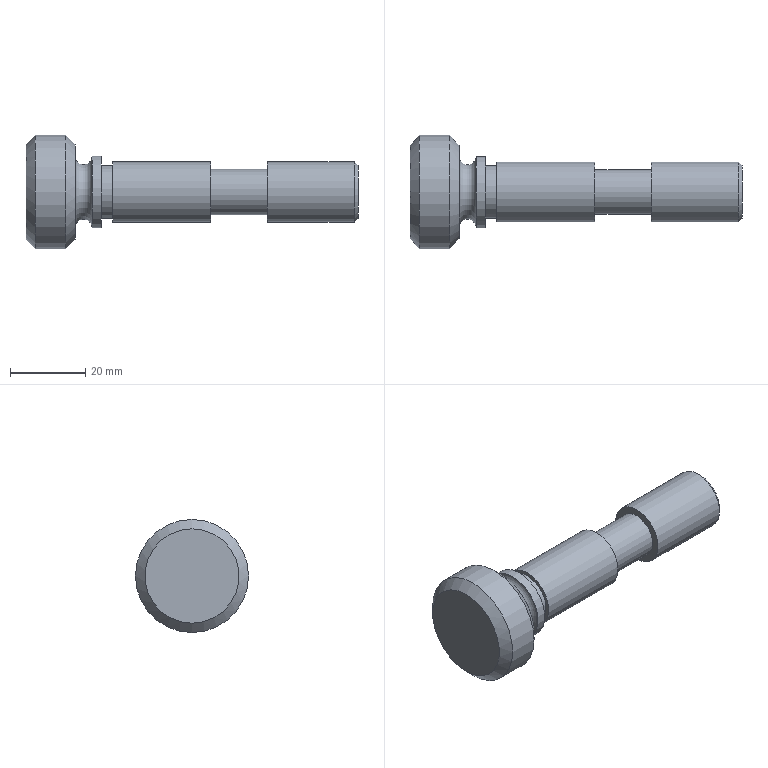Component | NX | SCREW_ROD | 1 solid | 17 faces | box 88 x 30 x 30 mm | volume 22378 mm3 | plane 7 | cylinder 6 | cone 3 | torus 1 | commonest cylinder face diameters 16 x2 12 x1 14 x1 19 x1 30 x1
STEP:
#1=CARTESIAN_POINT('',(0.,0.,0.));
#2=DIRECTION('',(0.,0.,1.));
#3=DIRECTION('',(1.,0.,0.));
#4=AXIS2_PLACEMENT_3D('',#1,#2,#3);
#5=CARTESIAN_POINT('',(-29.415,0.,-12.5));
#6=VERTEX_POINT('',#5);
#7=CARTESIAN_POINT('',(-29.415,0.,0.));
#8=DIRECTION('',(1.,0.,0.));
#9=DIRECTION('',(0.,0.,-1.));
#10=AXIS2_PLACEMENT_3D('',#7,#8,#9);
#11=CIRCLE('',#10,12.5);
#12=CARTESIAN_POINT('',(-29.415,0.,0.));
#13=DIRECTION('',(1.,0.,0.));
#14=DIRECTION('',(0.,0.,-1.));
#15=AXIS2_PLACEMENT_3D('',#12,#13,#14);
#16=PLANE('',#15);
#17=CARTESIAN_POINT('',(0.,0.));
#18=DIRECTION('',(1.,0.));
#19=AXIS2_PLACEMENT_2D('',#17,#18);
#20=CIRCLE('',#19,12.5);
#21=(GEOMETRIC_REPRESENTATION_CONTEXT(2)PARAMETRIC_REPRESENTATION_CONTEXT()REPRESENTATION_CONTEXT('',''));
#22=DEFINITIONAL_REPRESENTATION('',(#20),#21);
#23=PCURVE('',#16,#22);
#24=CARTESIAN_POINT('',(-29.415,0.,0.));
#25=DIRECTION('',(1.,0.,0.));
#26=DIRECTION('',(0.,0.,-1.));
#27=AXIS2_PLACEMENT_3D('',#24,#25,#26);
#28=CONICAL_SURFACE('',#27,12.5,0.7854);
#29=CARTESIAN_POINT('',(0.,0.));
#30=DIRECTION('',(1.,0.));
#31=VECTOR('',#30,1.);
#32=LINE('',#29,#31);
#33=(GEOMETRIC_REPRESENTATION_CONTEXT(2)PARAMETRIC_REPRESENTATION_CONTEXT()REPRESENTATION_CONTEXT('',''));
#34=DEFINITIONAL_REPRESENTATION('',(#32),#33);
#35=PCURVE('',#28,#34);
#36=SURFACE_CURVE('',#11,(#23,#35),.PCURVE_S1.);
#37=EDGE_CURVE('',#6,#6,#36,.T.);
#38=ORIENTED_EDGE('',*,*,#37,.F.);
#39=EDGE_LOOP('',(#38));
#40=FACE_BOUND('',#39,.T.);
#41=ADVANCED_FACE('',(#40),#16,.F.);
#42=CARTESIAN_POINT('',(58.585,0.,-7.));
#43=VERTEX_POINT('',#42);
#44=CARTESIAN_POINT('',(58.585,0.,0.));
#45=DIRECTION('',(1.,0.,0.));
#46=DIRECTION('',(0.,0.,-1.));
#47=AXIS2_PLACEMENT_3D('',#44,#45,#46);
#48=CIRCLE('',#47,7.);
#49=CARTESIAN_POINT('',(58.585,0.,0.));
#50=DIRECTION('',(1.,0.,0.));
#51=DIRECTION('',(0.,0.,-1.));
#52=AXIS2_PLACEMENT_3D('',#49,#50,#51);
#53=PLANE('',#52);
#54=CARTESIAN_POINT('',(0.,0.));
#55=DIRECTION('',(1.,0.));
#56=AXIS2_PLACEMENT_2D('',#54,#55);
#57=CIRCLE('',#56,7.);
#58=(GEOMETRIC_REPRESENTATION_CONTEXT(2)PARAMETRIC_REPRESENTATION_CONTEXT()REPRESENTATION_CONTEXT('',''));
#59=DEFINITIONAL_REPRESENTATION('',(#57),#58);
#60=PCURVE('',#53,#59);
#61=CARTESIAN_POINT('',(58.585,0.,0.));
#62=DIRECTION('',(-1.,0.,0.));
#63=DIRECTION('',(0.,0.,1.));
#64=AXIS2_PLACEMENT_3D('',#61,#62,#63);
#65=CONICAL_SURFACE('',#64,7.,0.7854);
#66=CARTESIAN_POINT('',(9.425,0.));
#67=DIRECTION('',(-1.,0.));
#68=VECTOR('',#67,1.);
#69=LINE('',#66,#68);
#70=(GEOMETRIC_REPRESENTATION_CONTEXT(2)PARAMETRIC_REPRESENTATION_CONTEXT()REPRESENTATION_CONTEXT('',''));
#71=DEFINITIONAL_REPRESENTATION('',(#69),#70);
#72=PCURVE('',#65,#71);
#73=SURFACE_CURVE('',#48,(#60,#72),.PCURVE_S1.);
#74=EDGE_CURVE('',#43,#43,#73,.T.);
#75=ORIENTED_EDGE('',*,*,#74,.T.);
#76=EDGE_LOOP('',(#75));
#77=FACE_BOUND('',#76,.T.);
#78=ADVANCED_FACE('',(#77),#53,.T.);
#79=CARTESIAN_POINT('',(57.585,0.,-8.));
#80=VERTEX_POINT('',#79);
#81=CARTESIAN_POINT('',(57.585,0.,0.));
#82=DIRECTION('',(-1.,0.,0.));
#83=DIRECTION('',(0.,0.,-1.));
#84=AXIS2_PLACEMENT_3D('',#81,#82,#83);
#85=CIRCLE('',#84,8.);
#86=CARTESIAN_POINT('',(58.585,0.,0.));
#87=DIRECTION('',(1.,0.,0.));
#88=DIRECTION('',(0.,0.,-1.));
#89=AXIS2_PLACEMENT_3D('',#86,#87,#88);
#90=CYLINDRICAL_SURFACE('',#89,8.);
#91=CARTESIAN_POINT('',(6.283,-1.));
#92=DIRECTION('',(-1.,0.));
#93=VECTOR('',#92,1.);
#94=LINE('',#91,#93);
#95=(GEOMETRIC_REPRESENTATION_CONTEXT(2)PARAMETRIC_REPRESENTATION_CONTEXT()REPRESENTATION_CONTEXT('',''));
#96=DEFINITIONAL_REPRESENTATION('',(#94),#95);
#97=PCURVE('',#90,#96);
#98=CARTESIAN_POINT('',(3.142,1.));
#99=DIRECTION('',(1.,0.));
#100=VECTOR('',#99,1.);
#101=LINE('',#98,#100);
#102=(GEOMETRIC_REPRESENTATION_CONTEXT(2)PARAMETRIC_REPRESENTATION_CONTEXT()REPRESENTATION_CONTEXT('',''));
#103=DEFINITIONAL_REPRESENTATION('',(#101),#102);
#104=PCURVE('',#65,#103);
#105=SURFACE_CURVE('',#85,(#97,#104),.PCURVE_S1.);
#106=EDGE_CURVE('',#80,#80,#105,.T.);
#107=ORIENTED_EDGE('',*,*,#106,.T.);
#108=CARTESIAN_POINT('',(34.585,0.,-8.));
#109=VERTEX_POINT('',#108);
#110=CARTESIAN_POINT('',(34.585,-0.,-8.));
#111=CARTESIAN_POINT('',(57.585,-0.,-8.));
#112=B_SPLINE_CURVE_WITH_KNOTS('',1,(#110,#111),.UNSPECIFIED.,.F.,.F.,(2,2),(-24.,-1.),.PIECEWISE_BEZIER_KNOTS.);
#113=CARTESIAN_POINT('',(0.,0.));
#114=DIRECTION('',(0.,1.));
#115=VECTOR('',#114,1.);
#116=LINE('',#113,#115);
#117=(GEOMETRIC_REPRESENTATION_CONTEXT(2)PARAMETRIC_REPRESENTATION_CONTEXT()REPRESENTATION_CONTEXT('',''));
#118=DEFINITIONAL_REPRESENTATION('',(#116),#117);
#119=PCURVE('',#90,#118);
#120=CARTESIAN_POINT('',(6.283,0.));
#121=DIRECTION('',(0.,1.));
#122=VECTOR('',#121,1.);
#123=LINE('',#120,#122);
#124=(GEOMETRIC_REPRESENTATION_CONTEXT(2)PARAMETRIC_REPRESENTATION_CONTEXT()REPRESENTATION_CONTEXT('',''));
#125=DEFINITIONAL_REPRESENTATION('',(#123),#124);
#126=PCURVE('',#90,#125);
#127=SEAM_CURVE('',#112,(#119,#126),.PCURVE_S1.);
#128=EDGE_CURVE('',#109,#80,#127,.T.);
#129=ORIENTED_EDGE('',*,*,#128,.F.);
#130=CARTESIAN_POINT('',(34.585,0.,0.));
#131=DIRECTION('',(1.,0.,0.));
#132=DIRECTION('',(0.,0.,-1.));
#133=AXIS2_PLACEMENT_3D('',#130,#131,#132);
#134=CIRCLE('',#133,8.);
#135=CARTESIAN_POINT('',(0.,-24.));
#136=DIRECTION('',(1.,0.));
#137=VECTOR('',#136,1.);
#138=LINE('',#135,#137);
#139=(GEOMETRIC_REPRESENTATION_CONTEXT(2)PARAMETRIC_REPRESENTATION_CONTEXT()REPRESENTATION_CONTEXT('',''));
#140=DEFINITIONAL_REPRESENTATION('',(#138),#139);
#141=PCURVE('',#90,#140);
#142=CARTESIAN_POINT('',(34.585,6.,0.));
#143=DIRECTION('',(1.,0.,0.));
#144=DIRECTION('',(0.,0.,-1.));
#145=AXIS2_PLACEMENT_3D('',#142,#143,#144);
#146=PLANE('',#145);
#147=CARTESIAN_POINT('',(0.,-6.));
#148=DIRECTION('',(1.,0.));
#149=AXIS2_PLACEMENT_2D('',#147,#148);
#150=CIRCLE('',#149,8.);
#151=(GEOMETRIC_REPRESENTATION_CONTEXT(2)PARAMETRIC_REPRESENTATION_CONTEXT()REPRESENTATION_CONTEXT('',''));
#152=DEFINITIONAL_REPRESENTATION('',(#150),#151);
#153=PCURVE('',#146,#152);
#154=SURFACE_CURVE('',#134,(#141,#153),.PCURVE_S1.);
#155=EDGE_CURVE('',#109,#109,#154,.T.);
#156=ORIENTED_EDGE('',*,*,#155,.T.);
#157=ORIENTED_EDGE('',*,*,#128,.T.);
#158=EDGE_LOOP('',(#107,#129,#156,#157));
#159=FACE_BOUND('',#158,.T.);
#160=ADVANCED_FACE('',(#159),#90,.T.);
#161=ORIENTED_EDGE('',*,*,#155,.F.);
#162=EDGE_LOOP('',(#161));
#163=FACE_BOUND('',#162,.T.);
#164=CARTESIAN_POINT('',(34.585,0.,-6.));
#165=VERTEX_POINT('',#164);
#166=CARTESIAN_POINT('',(34.585,0.,0.));
#167=DIRECTION('',(1.,0.,0.));
#168=DIRECTION('',(0.,0.,-1.));
#169=AXIS2_PLACEMENT_3D('',#166,#167,#168);
#170=CIRCLE('',#169,6.);
#171=CARTESIAN_POINT('',(0.,-6.));
#172=DIRECTION('',(1.,0.));
#173=AXIS2_PLACEMENT_2D('',#171,#172);
#174=CIRCLE('',#173,6.);
#175=(GEOMETRIC_REPRESENTATION_CONTEXT(2)PARAMETRIC_REPRESENTATION_CONTEXT()REPRESENTATION_CONTEXT('',''));
#176=DEFINITIONAL_REPRESENTATION('',(#174),#175);
#177=PCURVE('',#146,#176);
#178=CARTESIAN_POINT('',(58.585,0.,0.));
#179=DIRECTION('',(1.,0.,0.));
#180=DIRECTION('',(0.,0.,-1.));
#181=AXIS2_PLACEMENT_3D('',#178,#179,#180);
#182=CYLINDRICAL_SURFACE('',#181,6.);
#183=CARTESIAN_POINT('',(0.,-24.));
#184=DIRECTION('',(1.,0.));
#185=VECTOR('',#184,1.);
#186=LINE('',#183,#185);
#187=(GEOMETRIC_REPRESENTATION_CONTEXT(2)PARAMETRIC_REPRESENTATION_CONTEXT()REPRESENTATION_CONTEXT('',''));
#188=DEFINITIONAL_REPRESENTATION('',(#186),#187);
#189=PCURVE('',#182,#188);
#190=SURFACE_CURVE('',#170,(#177,#189),.PCURVE_S1.);
#191=EDGE_CURVE('',#165,#165,#190,.T.);
#192=ORIENTED_EDGE('',*,*,#191,.T.);
#193=EDGE_LOOP('',(#192));
#194=FACE_BOUND('',#193,.T.);
#195=ADVANCED_FACE('',(#163,#194),#146,.F.);
#196=ORIENTED_EDGE('',*,*,#191,.F.);
#197=CARTESIAN_POINT('',(19.585,0.,-6.));
#198=VERTEX_POINT('',#197);
#199=CARTESIAN_POINT('',(19.585,-0.,-6.));
#200=CARTESIAN_POINT('',(34.585,-0.,-6.));
#201=B_SPLINE_CURVE_WITH_KNOTS('',1,(#199,#200),.UNSPECIFIED.,.F.,.F.,(2,2),(-39.,-24.),.PIECEWISE_BEZIER_KNOTS.);
#202=CARTESIAN_POINT('',(0.,0.));
#203=DIRECTION('',(0.,1.));
#204=VECTOR('',#203,1.);
#205=LINE('',#202,#204);
#206=(GEOMETRIC_REPRESENTATION_CONTEXT(2)PARAMETRIC_REPRESENTATION_CONTEXT()REPRESENTATION_CONTEXT('',''));
#207=DEFINITIONAL_REPRESENTATION('',(#205),#206);
#208=PCURVE('',#182,#207);
#209=CARTESIAN_POINT('',(6.283,0.));
#210=DIRECTION('',(0.,1.));
#211=VECTOR('',#210,1.);
#212=LINE('',#209,#211);
#213=(GEOMETRIC_REPRESENTATION_CONTEXT(2)PARAMETRIC_REPRESENTATION_CONTEXT()REPRESENTATION_CONTEXT('',''));
#214=DEFINITIONAL_REPRESENTATION('',(#212),#213);
#215=PCURVE('',#182,#214);
#216=SEAM_CURVE('',#201,(#208,#215),.PCURVE_S1.);
#217=EDGE_CURVE('',#198,#165,#216,.T.);
#218=ORIENTED_EDGE('',*,*,#217,.F.);
#219=CARTESIAN_POINT('',(19.585,0.,0.));
#220=DIRECTION('',(1.,0.,0.));
#221=DIRECTION('',(0.,0.,-1.));
#222=AXIS2_PLACEMENT_3D('',#219,#220,#221);
#223=CIRCLE('',#222,6.);
#224=CARTESIAN_POINT('',(0.,-39.));
#225=DIRECTION('',(1.,0.));
#226=VECTOR('',#225,1.);
#227=LINE('',#224,#226);
#228=(GEOMETRIC_REPRESENTATION_CONTEXT(2)PARAMETRIC_REPRESENTATION_CONTEXT()REPRESENTATION_CONTEXT('',''));
#229=DEFINITIONAL_REPRESENTATION('',(#227),#228);
#230=PCURVE('',#182,#229);
#231=CARTESIAN_POINT('',(19.585,8.,0.));
#232=DIRECTION('',(-1.,0.,0.));
#233=DIRECTION('',(0.,0.,1.));
#234=AXIS2_PLACEMENT_3D('',#231,#232,#233);
#235=PLANE('',#234);
#236=CARTESIAN_POINT('',(-6.,-8.));
#237=CARTESIAN_POINT('',(-6.,2.392));
#238=CARTESIAN_POINT('',(3.,-2.804));
#239=CARTESIAN_POINT('',(12.,-8.));
#240=CARTESIAN_POINT('',(3.,-13.196));
#241=CARTESIAN_POINT('',(-6.,-18.392));
#242=CARTESIAN_POINT('',(-6.,-8.));
#243=(BOUNDED_CURVE()B_SPLINE_CURVE(2,(#236,#237,#238,#239,#240,#241,#242),.UNSPECIFIED.,.T.,.F.)B_SPLINE_CURVE_WITH_KNOTS((1,2,2,2,2,1),(-2.094,0.,2.094,4.189,6.283,8.378),.UNSPECIFIED.)CURVE()GEOMETRIC_REPRESENTATION_ITEM()RATIONAL_B_SPLINE_CURVE((1.,0.5,1.,0.5,1.,0.5,1.))REPRESENTATION_ITEM(''));
#244=(GEOMETRIC_REPRESENTATION_CONTEXT(2)PARAMETRIC_REPRESENTATION_CONTEXT()REPRESENTATION_CONTEXT('',''));
#245=DEFINITIONAL_REPRESENTATION('',(#243),#244);
#246=PCURVE('',#235,#245);
#247=SURFACE_CURVE('',#223,(#230,#246),.PCURVE_S1.);
#248=EDGE_CURVE('',#198,#198,#247,.T.);
#249=ORIENTED_EDGE('',*,*,#248,.T.);
#250=ORIENTED_EDGE('',*,*,#217,.T.);
#251=EDGE_LOOP('',(#196,#218,#249,#250));
#252=FACE_BOUND('',#251,.T.);
#253=ADVANCED_FACE('',(#252),#182,.T.);
#254=ORIENTED_EDGE('',*,*,#248,.F.);
#255=EDGE_LOOP('',(#254));
#256=FACE_BOUND('',#255,.T.);
#257=CARTESIAN_POINT('',(19.585,0.,-8.));
#258=VERTEX_POINT('',#257);
#259=CARTESIAN_POINT('',(19.585,0.,0.));
#260=DIRECTION('',(1.,0.,0.));
#261=DIRECTION('',(0.,0.,-1.));
#262=AXIS2_PLACEMENT_3D('',#259,#260,#261);
#263=CIRCLE('',#262,8.);
#264=CARTESIAN_POINT('',(-8.,-8.));
#265=CARTESIAN_POINT('',(-8.,5.856));
#266=CARTESIAN_POINT('',(4.,-1.072));
#267=CARTESIAN_POINT('',(16.,-8.));
#268=CARTESIAN_POINT('',(4.,-14.928));
#269=CARTESIAN_POINT('',(-8.,-21.856));
#270=CARTESIAN_POINT('',(-8.,-8.));
#271=(BOUNDED_CURVE()B_SPLINE_CURVE(2,(#264,#265,#266,#267,#268,#269,#270),.UNSPECIFIED.,.T.,.F.)B_SPLINE_CURVE_WITH_KNOTS((1,2,2,2,2,1),(-2.094,0.,2.094,4.189,6.283,8.378),.UNSPECIFIED.)CURVE()GEOMETRIC_REPRESENTATION_ITEM()RATIONAL_B_SPLINE_CURVE((1.,0.5,1.,0.5,1.,0.5,1.))REPRESENTATION_ITEM(''));
#272=(GEOMETRIC_REPRESENTATION_CONTEXT(2)PARAMETRIC_REPRESENTATION_CONTEXT()REPRESENTATION_CONTEXT('',''));
#273=DEFINITIONAL_REPRESENTATION('',(#271),#272);
#274=PCURVE('',#235,#273);
#275=CARTESIAN_POINT('',(58.585,0.,0.));
#276=DIRECTION('',(1.,0.,0.));
#277=DIRECTION('',(0.,0.,-1.));
#278=AXIS2_PLACEMENT_3D('',#275,#276,#277);
#279=CYLINDRICAL_SURFACE('',#278,8.);
#280=CARTESIAN_POINT('',(0.,-39.));
#281=DIRECTION('',(1.,0.));
#282=VECTOR('',#281,1.);
#283=LINE('',#280,#282);
#284=(GEOMETRIC_REPRESENTATION_CONTEXT(2)PARAMETRIC_REPRESENTATION_CONTEXT()REPRESENTATION_CONTEXT('',''));
#285=DEFINITIONAL_REPRESENTATION('',(#283),#284);
#286=PCURVE('',#279,#285);
#287=SURFACE_CURVE('',#263,(#274,#286),.PCURVE_S1.);
#288=EDGE_CURVE('',#258,#258,#287,.T.);
#289=ORIENTED_EDGE('',*,*,#288,.T.);
#290=EDGE_LOOP('',(#289));
#291=FACE_BOUND('',#290,.T.);
#292=ADVANCED_FACE('',(#256,#291),#235,.F.);
#293=ORIENTED_EDGE('',*,*,#288,.F.);
#294=CARTESIAN_POINT('',(-6.415,0.,-8.));
#295=VERTEX_POINT('',#294);
#296=CARTESIAN_POINT('',(-6.415,-0.,-8.));
#297=CARTESIAN_POINT('',(19.585,-0.,-8.));
#298=B_SPLINE_CURVE_WITH_KNOTS('',1,(#296,#297),.UNSPECIFIED.,.F.,.F.,(2,2),(-65.,-39.),.PIECEWISE_BEZIER_KNOTS.);
#299=CARTESIAN_POINT('',(0.,0.));
#300=DIRECTION('',(0.,1.));
#301=VECTOR('',#300,1.);
#302=LINE('',#299,#301);
#303=(GEOMETRIC_REPRESENTATION_CONTEXT(2)PARAMETRIC_REPRESENTATION_CONTEXT()REPRESENTATION_CONTEXT('',''));
#304=DEFINITIONAL_REPRESENTATION('',(#302),#303);
#305=PCURVE('',#279,#304);
#306=CARTESIAN_POINT('',(6.283,0.));
#307=DIRECTION('',(0.,1.));
#308=VECTOR('',#307,1.);
#309=LINE('',#306,#308);
#310=(GEOMETRIC_REPRESENTATION_CONTEXT(2)PARAMETRIC_REPRESENTATION_CONTEXT()REPRESENTATION_CONTEXT('',''));
#311=DEFINITIONAL_REPRESENTATION('',(#309),#310);
#312=PCURVE('',#279,#311);
#313=SEAM_CURVE('',#298,(#305,#312),.PCURVE_S1.);
#314=EDGE_CURVE('',#295,#258,#313,.T.);
#315=ORIENTED_EDGE('',*,*,#314,.F.);
#316=CARTESIAN_POINT('',(-6.415,0.,0.));
#317=DIRECTION('',(1.,0.,0.));
#318=DIRECTION('',(0.,0.,-1.));
#319=AXIS2_PLACEMENT_3D('',#316,#317,#318);
#320=CIRCLE('',#319,8.);
#321=CARTESIAN_POINT('',(0.,-65.));
#322=DIRECTION('',(1.,0.));
#323=VECTOR('',#322,1.);
#324=LINE('',#321,#323);
#325=(GEOMETRIC_REPRESENTATION_CONTEXT(2)PARAMETRIC_REPRESENTATION_CONTEXT()REPRESENTATION_CONTEXT('',''));
#326=DEFINITIONAL_REPRESENTATION('',(#324),#325);
#327=PCURVE('',#279,#326);
#328=CARTESIAN_POINT('',(-6.415,7.,0.));
#329=DIRECTION('',(1.,0.,0.));
#330=DIRECTION('',(0.,0.,-1.));
#331=AXIS2_PLACEMENT_3D('',#328,#329,#330);
#332=PLANE('',#331);
#333=CARTESIAN_POINT('',(0.,-7.));
#334=DIRECTION('',(1.,0.));
#335=AXIS2_PLACEMENT_2D('',#333,#334);
#336=CIRCLE('',#335,8.);
#337=(GEOMETRIC_REPRESENTATION_CONTEXT(2)PARAMETRIC_REPRESENTATION_CONTEXT()REPRESENTATION_CONTEXT('',''));
#338=DEFINITIONAL_REPRESENTATION('',(#336),#337);
#339=PCURVE('',#332,#338);
#340=SURFACE_CURVE('',#320,(#327,#339),.PCURVE_S1.);
#341=EDGE_CURVE('',#295,#295,#340,.T.);
#342=ORIENTED_EDGE('',*,*,#341,.T.);
#343=ORIENTED_EDGE('',*,*,#314,.T.);
#344=EDGE_LOOP('',(#293,#315,#342,#343));
#345=FACE_BOUND('',#344,.T.);
#346=ADVANCED_FACE('',(#345),#279,.T.);
#347=ORIENTED_EDGE('',*,*,#341,.F.);
#348=EDGE_LOOP('',(#347));
#349=FACE_BOUND('',#348,.T.);
#350=CARTESIAN_POINT('',(-6.415,0.,-7.));
#351=VERTEX_POINT('',#350);
#352=CARTESIAN_POINT('',(-6.415,0.,0.));
#353=DIRECTION('',(1.,0.,0.));
#354=DIRECTION('',(0.,0.,-1.));
#355=AXIS2_PLACEMENT_3D('',#352,#353,#354);
#356=CIRCLE('',#355,7.);
#357=CARTESIAN_POINT('',(0.,-7.));
#358=DIRECTION('',(1.,0.));
#359=AXIS2_PLACEMENT_2D('',#357,#358);
#360=CIRCLE('',#359,7.);
#361=(GEOMETRIC_REPRESENTATION_CONTEXT(2)PARAMETRIC_REPRESENTATION_CONTEXT()REPRESENTATION_CONTEXT('',''));
#362=DEFINITIONAL_REPRESENTATION('',(#360),#361);
#363=PCURVE('',#332,#362);
#364=CARTESIAN_POINT('',(58.585,0.,0.));
#365=DIRECTION('',(1.,0.,0.));
#366=DIRECTION('',(0.,0.,-1.));
#367=AXIS2_PLACEMENT_3D('',#364,#365,#366);
#368=CYLINDRICAL_SURFACE('',#367,7.);
#369=CARTESIAN_POINT('',(0.,-65.));
#370=DIRECTION('',(1.,0.));
#371=VECTOR('',#370,1.);
#372=LINE('',#369,#371);
#373=(GEOMETRIC_REPRESENTATION_CONTEXT(2)PARAMETRIC_REPRESENTATION_CONTEXT()REPRESENTATION_CONTEXT('',''));
#374=DEFINITIONAL_REPRESENTATION('',(#372),#373);
#375=PCURVE('',#368,#374);
#376=SURFACE_CURVE('',#356,(#363,#375),.PCURVE_S1.);
#377=EDGE_CURVE('',#351,#351,#376,.T.);
#378=ORIENTED_EDGE('',*,*,#377,.T.);
#379=EDGE_LOOP('',(#378));
#380=FACE_BOUND('',#379,.T.);
#381=ADVANCED_FACE('',(#349,#380),#332,.F.);
#382=ORIENTED_EDGE('',*,*,#377,.F.);
#383=CARTESIAN_POINT('',(-9.415,0.,-7.));
#384=VERTEX_POINT('',#383);
#385=CARTESIAN_POINT('',(-9.415,-0.,-7.));
#386=CARTESIAN_POINT('',(-6.415,-0.,-7.));
#387=B_SPLINE_CURVE_WITH_KNOTS('',1,(#385,#386),.UNSPECIFIED.,.F.,.F.,(2,2),(-68.,-65.),.PIECEWISE_BEZIER_KNOTS.);
#388=CARTESIAN_POINT('',(0.,0.));
#389=DIRECTION('',(0.,1.));
#390=VECTOR('',#389,1.);
#391=LINE('',#388,#390);
#392=(GEOMETRIC_REPRESENTATION_CONTEXT(2)PARAMETRIC_REPRESENTATION_CONTEXT()REPRESENTATION_CONTEXT('',''));
#393=DEFINITIONAL_REPRESENTATION('',(#391),#392);
#394=PCURVE('',#368,#393);
#395=CARTESIAN_POINT('',(6.283,0.));
#396=DIRECTION('',(0.,1.));
#397=VECTOR('',#396,1.);
#398=LINE('',#395,#397);
#399=(GEOMETRIC_REPRESENTATION_CONTEXT(2)PARAMETRIC_REPRESENTATION_CONTEXT()REPRESENTATION_CONTEXT('',''));
#400=DEFINITIONAL_REPRESENTATION('',(#398),#399);
#401=PCURVE('',#368,#400);
#402=SEAM_CURVE('',#387,(#394,#401),.PCURVE_S1.);
#403=EDGE_CURVE('',#384,#351,#402,.T.);
#404=ORIENTED_EDGE('',*,*,#403,.F.);
#405=CARTESIAN_POINT('',(-9.415,0.,0.));
#406=DIRECTION('',(1.,0.,0.));
#407=DIRECTION('',(0.,0.,-1.));
#408=AXIS2_PLACEMENT_3D('',#405,#406,#407);
#409=CIRCLE('',#408,7.);
#410=CARTESIAN_POINT('',(0.,-68.));
#411=DIRECTION('',(1.,0.));
#412=VECTOR('',#411,1.);
#413=LINE('',#410,#412);
#414=(GEOMETRIC_REPRESENTATION_CONTEXT(2)PARAMETRIC_REPRESENTATION_CONTEXT()REPRESENTATION_CONTEXT('',''));
#415=DEFINITIONAL_REPRESENTATION('',(#413),#414);
#416=PCURVE('',#368,#415);
#417=CARTESIAN_POINT('',(-9.415,9.5,0.));
#418=DIRECTION('',(-1.,0.,0.));
#419=DIRECTION('',(0.,0.,1.));
#420=AXIS2_PLACEMENT_3D('',#417,#418,#419);
#421=PLANE('',#420);
#422=CARTESIAN_POINT('',(-7.,-9.5));
#423=CARTESIAN_POINT('',(-7.,2.624));
#424=CARTESIAN_POINT('',(3.5,-3.438));
#425=CARTESIAN_POINT('',(14.,-9.5));
#426=CARTESIAN_POINT('',(3.5,-15.562));
#427=CARTESIAN_POINT('',(-7.,-21.624));
#428=CARTESIAN_POINT('',(-7.,-9.5));
#429=(BOUNDED_CURVE()B_SPLINE_CURVE(2,(#422,#423,#424,#425,#426,#427,#428),.UNSPECIFIED.,.T.,.F.)B_SPLINE_CURVE_WITH_KNOTS((1,2,2,2,2,1),(-2.094,0.,2.094,4.189,6.283,8.378),.UNSPECIFIED.)CURVE()GEOMETRIC_REPRESENTATION_ITEM()RATIONAL_B_SPLINE_CURVE((1.,0.5,1.,0.5,1.,0.5,1.))REPRESENTATION_ITEM(''));
#430=(GEOMETRIC_REPRESENTATION_CONTEXT(2)PARAMETRIC_REPRESENTATION_CONTEXT()REPRESENTATION_CONTEXT('',''));
#431=DEFINITIONAL_REPRESENTATION('',(#429),#430);
#432=PCURVE('',#421,#431);
#433=SURFACE_CURVE('',#409,(#416,#432),.PCURVE_S1.);
#434=EDGE_CURVE('',#384,#384,#433,.T.);
#435=ORIENTED_EDGE('',*,*,#434,.T.);
#436=ORIENTED_EDGE('',*,*,#403,.T.);
#437=EDGE_LOOP('',(#382,#404,#435,#436));
#438=FACE_BOUND('',#437,.T.);
#439=ADVANCED_FACE('',(#438),#368,.T.);
#440=ORIENTED_EDGE('',*,*,#434,.F.);
#441=EDGE_LOOP('',(#440));
#442=FACE_BOUND('',#441,.T.);
#443=CARTESIAN_POINT('',(-9.415,0.,-9.5));
#444=VERTEX_POINT('',#443);
#445=CARTESIAN_POINT('',(-9.415,0.,0.));
#446=DIRECTION('',(1.,0.,0.));
#447=DIRECTION('',(0.,0.,-1.));
#448=AXIS2_PLACEMENT_3D('',#445,#446,#447);
#449=CIRCLE('',#448,9.5);
#450=CARTESIAN_POINT('',(-9.5,-9.5));
#451=CARTESIAN_POINT('',(-9.5,6.954));
#452=CARTESIAN_POINT('',(4.75,-1.273));
#453=CARTESIAN_POINT('',(19.,-9.5));
#454=CARTESIAN_POINT('',(4.75,-17.727));
#455=CARTESIAN_POINT('',(-9.5,-25.954));
#456=CARTESIAN_POINT('',(-9.5,-9.5));
#457=(BOUNDED_CURVE()B_SPLINE_CURVE(2,(#450,#451,#452,#453,#454,#455,#456),.UNSPECIFIED.,.T.,.F.)B_SPLINE_CURVE_WITH_KNOTS((1,2,2,2,2,1),(-2.094,0.,2.094,4.189,6.283,8.378),.UNSPECIFIED.)CURVE()GEOMETRIC_REPRESENTATION_ITEM()RATIONAL_B_SPLINE_CURVE((1.,0.5,1.,0.5,1.,0.5,1.))REPRESENTATION_ITEM(''));
#458=(GEOMETRIC_REPRESENTATION_CONTEXT(2)PARAMETRIC_REPRESENTATION_CONTEXT()REPRESENTATION_CONTEXT('',''));
#459=DEFINITIONAL_REPRESENTATION('',(#457),#458);
#460=PCURVE('',#421,#459);
#461=CARTESIAN_POINT('',(58.585,0.,0.));
#462=DIRECTION('',(1.,0.,0.));
#463=DIRECTION('',(0.,0.,-1.));
#464=AXIS2_PLACEMENT_3D('',#461,#462,#463);
#465=CYLINDRICAL_SURFACE('',#464,9.5);
#466=CARTESIAN_POINT('',(0.,-68.));
#467=DIRECTION('',(1.,0.));
#468=VECTOR('',#467,1.);
#469=LINE('',#466,#468);
#470=(GEOMETRIC_REPRESENTATION_CONTEXT(2)PARAMETRIC_REPRESENTATION_CONTEXT()REPRESENTATION_CONTEXT('',''));
#471=DEFINITIONAL_REPRESENTATION('',(#469),#470);
#472=PCURVE('',#465,#471);
#473=SURFACE_CURVE('',#449,(#460,#472),.PCURVE_S1.);
#474=EDGE_CURVE('',#444,#444,#473,.T.);
#475=ORIENTED_EDGE('',*,*,#474,.T.);
#476=EDGE_LOOP('',(#475));
#477=FACE_BOUND('',#476,.T.);
#478=ADVANCED_FACE('',(#442,#477),#421,.F.);
#479=ORIENTED_EDGE('',*,*,#474,.F.);
#480=CARTESIAN_POINT('',(-11.915,0.,-9.5));
#481=VERTEX_POINT('',#480);
#482=CARTESIAN_POINT('',(-11.915,-0.,-9.5));
#483=CARTESIAN_POINT('',(-9.415,-0.,-9.5));
#484=B_SPLINE_CURVE_WITH_KNOTS('',1,(#482,#483),.UNSPECIFIED.,.F.,.F.,(2,2),(-70.5,-68.),.PIECEWISE_BEZIER_KNOTS.);
#485=CARTESIAN_POINT('',(0.,0.));
#486=DIRECTION('',(0.,1.));
#487=VECTOR('',#486,1.);
#488=LINE('',#485,#487);
#489=(GEOMETRIC_REPRESENTATION_CONTEXT(2)PARAMETRIC_REPRESENTATION_CONTEXT()REPRESENTATION_CONTEXT('',''));
#490=DEFINITIONAL_REPRESENTATION('',(#488),#489);
#491=PCURVE('',#465,#490);
#492=CARTESIAN_POINT('',(6.283,0.));
#493=DIRECTION('',(0.,1.));
#494=VECTOR('',#493,1.);
#495=LINE('',#492,#494);
#496=(GEOMETRIC_REPRESENTATION_CONTEXT(2)PARAMETRIC_REPRESENTATION_CONTEXT()REPRESENTATION_CONTEXT('',''));
#497=DEFINITIONAL_REPRESENTATION('',(#495),#496);
#498=PCURVE('',#465,#497);
#499=SEAM_CURVE('',#484,(#491,#498),.PCURVE_S1.);
#500=EDGE_CURVE('',#481,#444,#499,.T.);
#501=ORIENTED_EDGE('',*,*,#500,.F.);
#502=CARTESIAN_POINT('',(-11.915,0.,0.));
#503=DIRECTION('',(1.,0.,0.));
#504=DIRECTION('',(0.,0.,-1.));
#505=AXIS2_PLACEMENT_3D('',#502,#503,#504);
#506=CIRCLE('',#505,9.5);
#507=CARTESIAN_POINT('',(0.,-70.5));
#508=DIRECTION('',(1.,0.));
#509=VECTOR('',#508,1.);
#510=LINE('',#507,#509);
#511=(GEOMETRIC_REPRESENTATION_CONTEXT(2)PARAMETRIC_REPRESENTATION_CONTEXT()REPRESENTATION_CONTEXT('',''));
#512=DEFINITIONAL_REPRESENTATION('',(#510),#511);
#513=PCURVE('',#465,#512);
#514=CARTESIAN_POINT('',(-14.165,0.,0.));
#515=DIRECTION('',(1.,0.,0.));
#516=DIRECTION('',(0.,0.,-1.));
#517=AXIS2_PLACEMENT_3D('',#514,#515,#516);
#518=TOROIDAL_SURFACE('',#517,9.5,2.25);
#519=CARTESIAN_POINT('',(0.,1.571));
#520=DIRECTION('',(1.,0.));
#521=VECTOR('',#520,1.);
#522=LINE('',#519,#521);
#523=(GEOMETRIC_REPRESENTATION_CONTEXT(2)PARAMETRIC_REPRESENTATION_CONTEXT()REPRESENTATION_CONTEXT('',''));
#524=DEFINITIONAL_REPRESENTATION('',(#522),#523);
#525=PCURVE('',#518,#524);
#526=SURFACE_CURVE('',#506,(#513,#525),.PCURVE_S1.);
#527=EDGE_CURVE('',#481,#481,#526,.T.);
#528=ORIENTED_EDGE('',*,*,#527,.T.);
#529=ORIENTED_EDGE('',*,*,#500,.T.);
#530=EDGE_LOOP('',(#479,#501,#528,#529));
#531=FACE_BOUND('',#530,.T.);
#532=ADVANCED_FACE('',(#531),#465,.T.);
#533=ORIENTED_EDGE('',*,*,#527,.T.);
#534=CARTESIAN_POINT('',(-16.415,0.,-9.5));
#535=VERTEX_POINT('',#534);
#536=CARTESIAN_POINT('',(-11.915,0.,-9.5));
#537=CARTESIAN_POINT('',(-11.915,0.,-8.616));
#538=CARTESIAN_POINT('',(-12.311,0.,-7.733));
#539=CARTESIAN_POINT('',(-13.104,0.,-7.057));
#540=CARTESIAN_POINT('',(-14.165,0.,-6.796));
#541=CARTESIAN_POINT('',(-15.225,0.,-7.057));
#542=CARTESIAN_POINT('',(-16.018,0.,-7.733));
#543=CARTESIAN_POINT('',(-16.415,0.,-8.616));
#544=CARTESIAN_POINT('',(-16.415,0.,-9.5));
#545=B_SPLINE_CURVE_WITH_KNOTS('',8,(#536,#537,#538,#539,#540,#541,#542,#543,#544),.UNSPECIFIED.,.F.,.F.,(9,9),(1.571,4.712),.PIECEWISE_BEZIER_KNOTS.);
#546=CARTESIAN_POINT('',(6.283,0.));
#547=DIRECTION('',(0.,1.));
#548=VECTOR('',#547,1.);
#549=LINE('',#546,#548);
#550=(GEOMETRIC_REPRESENTATION_CONTEXT(2)PARAMETRIC_REPRESENTATION_CONTEXT()REPRESENTATION_CONTEXT('',''));
#551=DEFINITIONAL_REPRESENTATION('',(#549),#550);
#552=PCURVE('',#518,#551);
#553=CARTESIAN_POINT('',(0.,0.));
#554=DIRECTION('',(0.,1.));
#555=VECTOR('',#554,1.);
#556=LINE('',#553,#555);
#557=(GEOMETRIC_REPRESENTATION_CONTEXT(2)PARAMETRIC_REPRESENTATION_CONTEXT()REPRESENTATION_CONTEXT('',''));
#558=DEFINITIONAL_REPRESENTATION('',(#556),#557);
#559=PCURVE('',#518,#558);
#560=SEAM_CURVE('',#545,(#552,#559),.PCURVE_S1.);
#561=EDGE_CURVE('',#481,#535,#560,.T.);
#562=ORIENTED_EDGE('',*,*,#561,.T.);
#563=CARTESIAN_POINT('',(-16.415,0.,0.));
#564=DIRECTION('',(1.,0.,0.));
#565=DIRECTION('',(0.,0.,-1.));
#566=AXIS2_PLACEMENT_3D('',#563,#564,#565);
#567=CIRCLE('',#566,9.5);
#568=CARTESIAN_POINT('',(0.,4.712));
#569=DIRECTION('',(1.,0.));
#570=VECTOR('',#569,1.);
#571=LINE('',#568,#570);
#572=(GEOMETRIC_REPRESENTATION_CONTEXT(2)PARAMETRIC_REPRESENTATION_CONTEXT()REPRESENTATION_CONTEXT('',''));
#573=DEFINITIONAL_REPRESENTATION('',(#571),#572);
#574=PCURVE('',#518,#573);
#575=CARTESIAN_POINT('',(-16.415,12.5,0.));
#576=DIRECTION('',(-1.,0.,0.));
#577=DIRECTION('',(0.,0.,1.));
#578=AXIS2_PLACEMENT_3D('',#575,#576,#577);
#579=PLANE('',#578);
#580=CARTESIAN_POINT('',(-9.5,-12.5));
#581=CARTESIAN_POINT('',(-9.5,3.954));
#582=CARTESIAN_POINT('',(4.75,-4.273));
#583=CARTESIAN_POINT('',(19.,-12.5));
#584=CARTESIAN_POINT('',(4.75,-20.727));
#585=CARTESIAN_POINT('',(-9.5,-28.954));
#586=CARTESIAN_POINT('',(-9.5,-12.5));
#587=(BOUNDED_CURVE()B_SPLINE_CURVE(2,(#580,#581,#582,#583,#584,#585,#586),.UNSPECIFIED.,.T.,.F.)B_SPLINE_CURVE_WITH_KNOTS((1,2,2,2,2,1),(-2.094,0.,2.094,4.189,6.283,8.378),.UNSPECIFIED.)CURVE()GEOMETRIC_REPRESENTATION_ITEM()RATIONAL_B_SPLINE_CURVE((1.,0.5,1.,0.5,1.,0.5,1.))REPRESENTATION_ITEM(''));
#588=(GEOMETRIC_REPRESENTATION_CONTEXT(2)PARAMETRIC_REPRESENTATION_CONTEXT()REPRESENTATION_CONTEXT('',''));
#589=DEFINITIONAL_REPRESENTATION('',(#587),#588);
#590=PCURVE('',#579,#589);
#591=SURFACE_CURVE('',#567,(#574,#590),.PCURVE_S1.);
#592=EDGE_CURVE('',#535,#535,#591,.T.);
#593=ORIENTED_EDGE('',*,*,#592,.F.);
#594=ORIENTED_EDGE('',*,*,#561,.F.);
#595=EDGE_LOOP('',(#533,#562,#593,#594));
#596=FACE_BOUND('',#595,.F.);
#597=ADVANCED_FACE('',(#596),#518,.F.);
#598=ORIENTED_EDGE('',*,*,#592,.F.);
#599=EDGE_LOOP('',(#598));
#600=FACE_BOUND('',#599,.T.);
#601=CARTESIAN_POINT('',(-16.415,0.,-12.5));
#602=VERTEX_POINT('',#601);
#603=CARTESIAN_POINT('',(-16.415,0.,0.));
#604=DIRECTION('',(1.,0.,0.));
#605=DIRECTION('',(0.,0.,-1.));
#606=AXIS2_PLACEMENT_3D('',#603,#604,#605);
#607=CIRCLE('',#606,12.5);
#608=CARTESIAN_POINT('',(-12.5,-12.5));
#609=CARTESIAN_POINT('',(-12.5,9.151));
#610=CARTESIAN_POINT('',(6.25,-1.675));
#611=CARTESIAN_POINT('',(25.,-12.5));
#612=CARTESIAN_POINT('',(6.25,-23.325));
#613=CARTESIAN_POINT('',(-12.5,-34.151));
#614=CARTESIAN_POINT('',(-12.5,-12.5));
#615=(BOUNDED_CURVE()B_SPLINE_CURVE(2,(#608,#609,#610,#611,#612,#613,#614),.UNSPECIFIED.,.T.,.F.)B_SPLINE_CURVE_WITH_KNOTS((1,2,2,2,2,1),(-2.094,0.,2.094,4.189,6.283,8.378),.UNSPECIFIED.)CURVE()GEOMETRIC_REPRESENTATION_ITEM()RATIONAL_B_SPLINE_CURVE((1.,0.5,1.,0.5,1.,0.5,1.))REPRESENTATION_ITEM(''));
#616=(GEOMETRIC_REPRESENTATION_CONTEXT(2)PARAMETRIC_REPRESENTATION_CONTEXT()REPRESENTATION_CONTEXT('',''));
#617=DEFINITIONAL_REPRESENTATION('',(#615),#616);
#618=PCURVE('',#579,#617);
#619=CARTESIAN_POINT('',(-18.915,0.,0.));
#620=DIRECTION('',(-1.,0.,0.));
#621=DIRECTION('',(0.,0.,1.));
#622=AXIS2_PLACEMENT_3D('',#619,#620,#621);
#623=CONICAL_SURFACE('',#622,15.,0.7854);
#624=CARTESIAN_POINT('',(9.425,-2.5));
#625=DIRECTION('',(-1.,0.));
#626=VECTOR('',#625,1.);
#627=LINE('',#624,#626);
#628=(GEOMETRIC_REPRESENTATION_CONTEXT(2)PARAMETRIC_REPRESENTATION_CONTEXT()REPRESENTATION_CONTEXT('',''));
#629=DEFINITIONAL_REPRESENTATION('',(#627),#628);
#630=PCURVE('',#623,#629);
#631=SURFACE_CURVE('',#607,(#618,#630),.PCURVE_S1.);
#632=EDGE_CURVE('',#602,#602,#631,.T.);
#633=ORIENTED_EDGE('',*,*,#632,.T.);
#634=EDGE_LOOP('',(#633));
#635=FACE_BOUND('',#634,.T.);
#636=ADVANCED_FACE('',(#600,#635),#579,.F.);
#637=ORIENTED_EDGE('',*,*,#632,.F.);
#638=CARTESIAN_POINT('',(-18.915,0.,-15.));
#639=VERTEX_POINT('',#638);
#640=CARTESIAN_POINT('',(-16.415,0.,-12.5));
#641=CARTESIAN_POINT('',(-18.915,0.,-15.));
#642=B_SPLINE_CURVE_WITH_KNOTS('',1,(#640,#641),.UNSPECIFIED.,.F.,.F.,(2,2),(-3.536,0.),.PIECEWISE_BEZIER_KNOTS.);
#643=CARTESIAN_POINT('',(9.425,0.));
#644=DIRECTION('',(0.,1.));
#645=VECTOR('',#644,1.);
#646=LINE('',#643,#645);
#647=(GEOMETRIC_REPRESENTATION_CONTEXT(2)PARAMETRIC_REPRESENTATION_CONTEXT()REPRESENTATION_CONTEXT('',''));
#648=DEFINITIONAL_REPRESENTATION('',(#646),#647);
#649=PCURVE('',#623,#648);
#650=CARTESIAN_POINT('',(3.142,0.));
#651=DIRECTION('',(0.,1.));
#652=VECTOR('',#651,1.);
#653=LINE('',#650,#652);
#654=(GEOMETRIC_REPRESENTATION_CONTEXT(2)PARAMETRIC_REPRESENTATION_CONTEXT()REPRESENTATION_CONTEXT('',''));
#655=DEFINITIONAL_REPRESENTATION('',(#653),#654);
#656=PCURVE('',#623,#655);
#657=SEAM_CURVE('',#642,(#649,#656),.PCURVE_S1.);
#658=EDGE_CURVE('',#602,#639,#657,.T.);
#659=ORIENTED_EDGE('',*,*,#658,.T.);
#660=CARTESIAN_POINT('',(-18.915,0.,0.));
#661=DIRECTION('',(1.,0.,0.));
#662=DIRECTION('',(0.,0.,-1.));
#663=AXIS2_PLACEMENT_3D('',#660,#661,#662);
#664=CIRCLE('',#663,15.);
#665=CARTESIAN_POINT('',(9.425,0.));
#666=DIRECTION('',(-1.,0.));
#667=VECTOR('',#666,1.);
#668=LINE('',#665,#667);
#669=(GEOMETRIC_REPRESENTATION_CONTEXT(2)PARAMETRIC_REPRESENTATION_CONTEXT()REPRESENTATION_CONTEXT('',''));
#670=DEFINITIONAL_REPRESENTATION('',(#668),#669);
#671=PCURVE('',#623,#670);
#672=CARTESIAN_POINT('',(58.585,0.,0.));
#673=DIRECTION('',(1.,0.,0.));
#674=DIRECTION('',(0.,0.,-1.));
#675=AXIS2_PLACEMENT_3D('',#672,#673,#674);
#676=CYLINDRICAL_SURFACE('',#675,15.);
#677=CARTESIAN_POINT('',(0.,-77.5));
#678=DIRECTION('',(1.,0.));
#679=VECTOR('',#678,1.);
#680=LINE('',#677,#679);
#681=(GEOMETRIC_REPRESENTATION_CONTEXT(2)PARAMETRIC_REPRESENTATION_CONTEXT()REPRESENTATION_CONTEXT('',''));
#682=DEFINITIONAL_REPRESENTATION('',(#680),#681);
#683=PCURVE('',#676,#682);
#684=SURFACE_CURVE('',#664,(#671,#683),.PCURVE_S1.);
#685=EDGE_CURVE('',#639,#639,#684,.T.);
#686=ORIENTED_EDGE('',*,*,#685,.T.);
#687=ORIENTED_EDGE('',*,*,#658,.F.);
#688=EDGE_LOOP('',(#637,#659,#686,#687));
#689=FACE_BOUND('',#688,.T.);
#690=ADVANCED_FACE('',(#689),#623,.T.);
#691=ORIENTED_EDGE('',*,*,#685,.F.);
#692=CARTESIAN_POINT('',(-26.915,0.,-15.));
#693=VERTEX_POINT('',#692);
#694=CARTESIAN_POINT('',(-26.915,-0.,-15.));
#695=CARTESIAN_POINT('',(-18.915,-0.,-15.));
#696=B_SPLINE_CURVE_WITH_KNOTS('',1,(#694,#695),.UNSPECIFIED.,.F.,.F.,(2,2),(-85.5,-77.5),.PIECEWISE_BEZIER_KNOTS.);
#697=CARTESIAN_POINT('',(0.,0.));
#698=DIRECTION('',(0.,1.));
#699=VECTOR('',#698,1.);
#700=LINE('',#697,#699);
#701=(GEOMETRIC_REPRESENTATION_CONTEXT(2)PARAMETRIC_REPRESENTATION_CONTEXT()REPRESENTATION_CONTEXT('',''));
#702=DEFINITIONAL_REPRESENTATION('',(#700),#701);
#703=PCURVE('',#676,#702);
#704=CARTESIAN_POINT('',(6.283,0.));
#705=DIRECTION('',(0.,1.));
#706=VECTOR('',#705,1.);
#707=LINE('',#704,#706);
#708=(GEOMETRIC_REPRESENTATION_CONTEXT(2)PARAMETRIC_REPRESENTATION_CONTEXT()REPRESENTATION_CONTEXT('',''));
#709=DEFINITIONAL_REPRESENTATION('',(#707),#708);
#710=PCURVE('',#676,#709);
#711=SEAM_CURVE('',#696,(#703,#710),.PCURVE_S1.);
#712=EDGE_CURVE('',#693,#639,#711,.T.);
#713=ORIENTED_EDGE('',*,*,#712,.F.);
#714=CARTESIAN_POINT('',(-26.915,0.,0.));
#715=DIRECTION('',(1.,0.,0.));
#716=DIRECTION('',(0.,0.,-1.));
#717=AXIS2_PLACEMENT_3D('',#714,#715,#716);
#718=CIRCLE('',#717,15.);
#719=CARTESIAN_POINT('',(0.,-85.5));
#720=DIRECTION('',(1.,0.));
#721=VECTOR('',#720,1.);
#722=LINE('',#719,#721);
#723=(GEOMETRIC_REPRESENTATION_CONTEXT(2)PARAMETRIC_REPRESENTATION_CONTEXT()REPRESENTATION_CONTEXT('',''));
#724=DEFINITIONAL_REPRESENTATION('',(#722),#723);
#725=PCURVE('',#676,#724);
#726=CARTESIAN_POINT('',(0.,2.5));
#727=DIRECTION('',(1.,0.));
#728=VECTOR('',#727,1.);
#729=LINE('',#726,#728);
#730=(GEOMETRIC_REPRESENTATION_CONTEXT(2)PARAMETRIC_REPRESENTATION_CONTEXT()REPRESENTATION_CONTEXT('',''));
#731=DEFINITIONAL_REPRESENTATION('',(#729),#730);
#732=PCURVE('',#28,#731);
#733=SURFACE_CURVE('',#718,(#725,#732),.PCURVE_S1.);
#734=EDGE_CURVE('',#693,#693,#733,.T.);
#735=ORIENTED_EDGE('',*,*,#734,.T.);
#736=ORIENTED_EDGE('',*,*,#712,.T.);
#737=EDGE_LOOP('',(#691,#713,#735,#736));
#738=FACE_BOUND('',#737,.T.);
#739=ADVANCED_FACE('',(#738),#676,.T.);
#740=ORIENTED_EDGE('',*,*,#734,.F.);
#741=CARTESIAN_POINT('',(-29.415,-0.,-12.5));
#742=CARTESIAN_POINT('',(-26.915,-0.,-15.));
#743=B_SPLINE_CURVE_WITH_KNOTS('',1,(#741,#742),.UNSPECIFIED.,.F.,.F.,(2,2),(0.,3.536),.PIECEWISE_BEZIER_KNOTS.);
#744=CARTESIAN_POINT('',(0.,0.));
#745=DIRECTION('',(0.,1.));
#746=VECTOR('',#745,1.);
#747=LINE('',#744,#746);
#748=(GEOMETRIC_REPRESENTATION_CONTEXT(2)PARAMETRIC_REPRESENTATION_CONTEXT()REPRESENTATION_CONTEXT('',''));
#749=DEFINITIONAL_REPRESENTATION('',(#747),#748);
#750=PCURVE('',#28,#749);
#751=CARTESIAN_POINT('',(6.283,0.));
#752=DIRECTION('',(0.,1.));
#753=VECTOR('',#752,1.);
#754=LINE('',#751,#753);
#755=(GEOMETRIC_REPRESENTATION_CONTEXT(2)PARAMETRIC_REPRESENTATION_CONTEXT()REPRESENTATION_CONTEXT('',''));
#756=DEFINITIONAL_REPRESENTATION('',(#754),#755);
#757=PCURVE('',#28,#756);
#758=SEAM_CURVE('',#743,(#750,#757),.PCURVE_S1.);
#759=EDGE_CURVE('',#6,#693,#758,.T.);
#760=ORIENTED_EDGE('',*,*,#759,.F.);
#761=ORIENTED_EDGE('',*,*,#37,.T.);
#762=ORIENTED_EDGE('',*,*,#759,.T.);
#763=EDGE_LOOP('',(#740,#760,#761,#762));
#764=FACE_BOUND('',#763,.T.);
#765=ADVANCED_FACE('',(#764),#28,.T.);
#766=ORIENTED_EDGE('',*,*,#106,.F.);
#767=CARTESIAN_POINT('',(58.585,0.,-7.));
#768=CARTESIAN_POINT('',(57.585,0.,-8.));
#769=B_SPLINE_CURVE_WITH_KNOTS('',1,(#767,#768),.UNSPECIFIED.,.F.,.F.,(2,2),(0.,1.414),.PIECEWISE_BEZIER_KNOTS.);
#770=CARTESIAN_POINT('',(3.142,0.));
#771=DIRECTION('',(0.,1.));
#772=VECTOR('',#771,1.);
#773=LINE('',#770,#772);
#774=(GEOMETRIC_REPRESENTATION_CONTEXT(2)PARAMETRIC_REPRESENTATION_CONTEXT()REPRESENTATION_CONTEXT('',''));
#775=DEFINITIONAL_REPRESENTATION('',(#773),#774);
#776=PCURVE('',#65,#775);
#777=CARTESIAN_POINT('',(9.425,0.));
#778=DIRECTION('',(0.,1.));
#779=VECTOR('',#778,1.);
#780=LINE('',#777,#779);
#781=(GEOMETRIC_REPRESENTATION_CONTEXT(2)PARAMETRIC_REPRESENTATION_CONTEXT()REPRESENTATION_CONTEXT('',''));
#782=DEFINITIONAL_REPRESENTATION('',(#780),#781);
#783=PCURVE('',#65,#782);
#784=SEAM_CURVE('',#769,(#776,#783),.PCURVE_S1.);
#785=EDGE_CURVE('',#43,#80,#784,.T.);
#786=ORIENTED_EDGE('',*,*,#785,.F.);
#787=ORIENTED_EDGE('',*,*,#74,.F.);
#788=ORIENTED_EDGE('',*,*,#785,.T.);
#789=EDGE_LOOP('',(#766,#786,#787,#788));
#790=FACE_BOUND('',#789,.T.);
#791=ADVANCED_FACE('',(#790),#65,.T.);
#792=CLOSED_SHELL('',(#41,#78,#160,#195,#253,#292,#346,#381,#439,#478,#532,#597,#636,#690,#739,#765,#791));
#793=MANIFOLD_SOLID_BREP('',#792);
#794=(LENGTH_UNIT()NAMED_UNIT(*)SI_UNIT(.MILLI.,.METRE.));
#795=UNCERTAINTY_MEASURE_WITH_UNIT(LENGTH_MEASURE(0.00001),#794,'','');
#796=(NAMED_UNIT(*)PLANE_ANGLE_UNIT()SI_UNIT($,.RADIAN.));
#797=(NAMED_UNIT(*)SI_UNIT($,.STERADIAN.)SOLID_ANGLE_UNIT());
#798=(GEOMETRIC_REPRESENTATION_CONTEXT(3)GLOBAL_UNCERTAINTY_ASSIGNED_CONTEXT((#795))GLOBAL_UNIT_ASSIGNED_CONTEXT((#794,#796,#797))REPRESENTATION_CONTEXT('',''));
#799=ADVANCED_BREP_SHAPE_REPRESENTATION('',(#4,#793),#798);